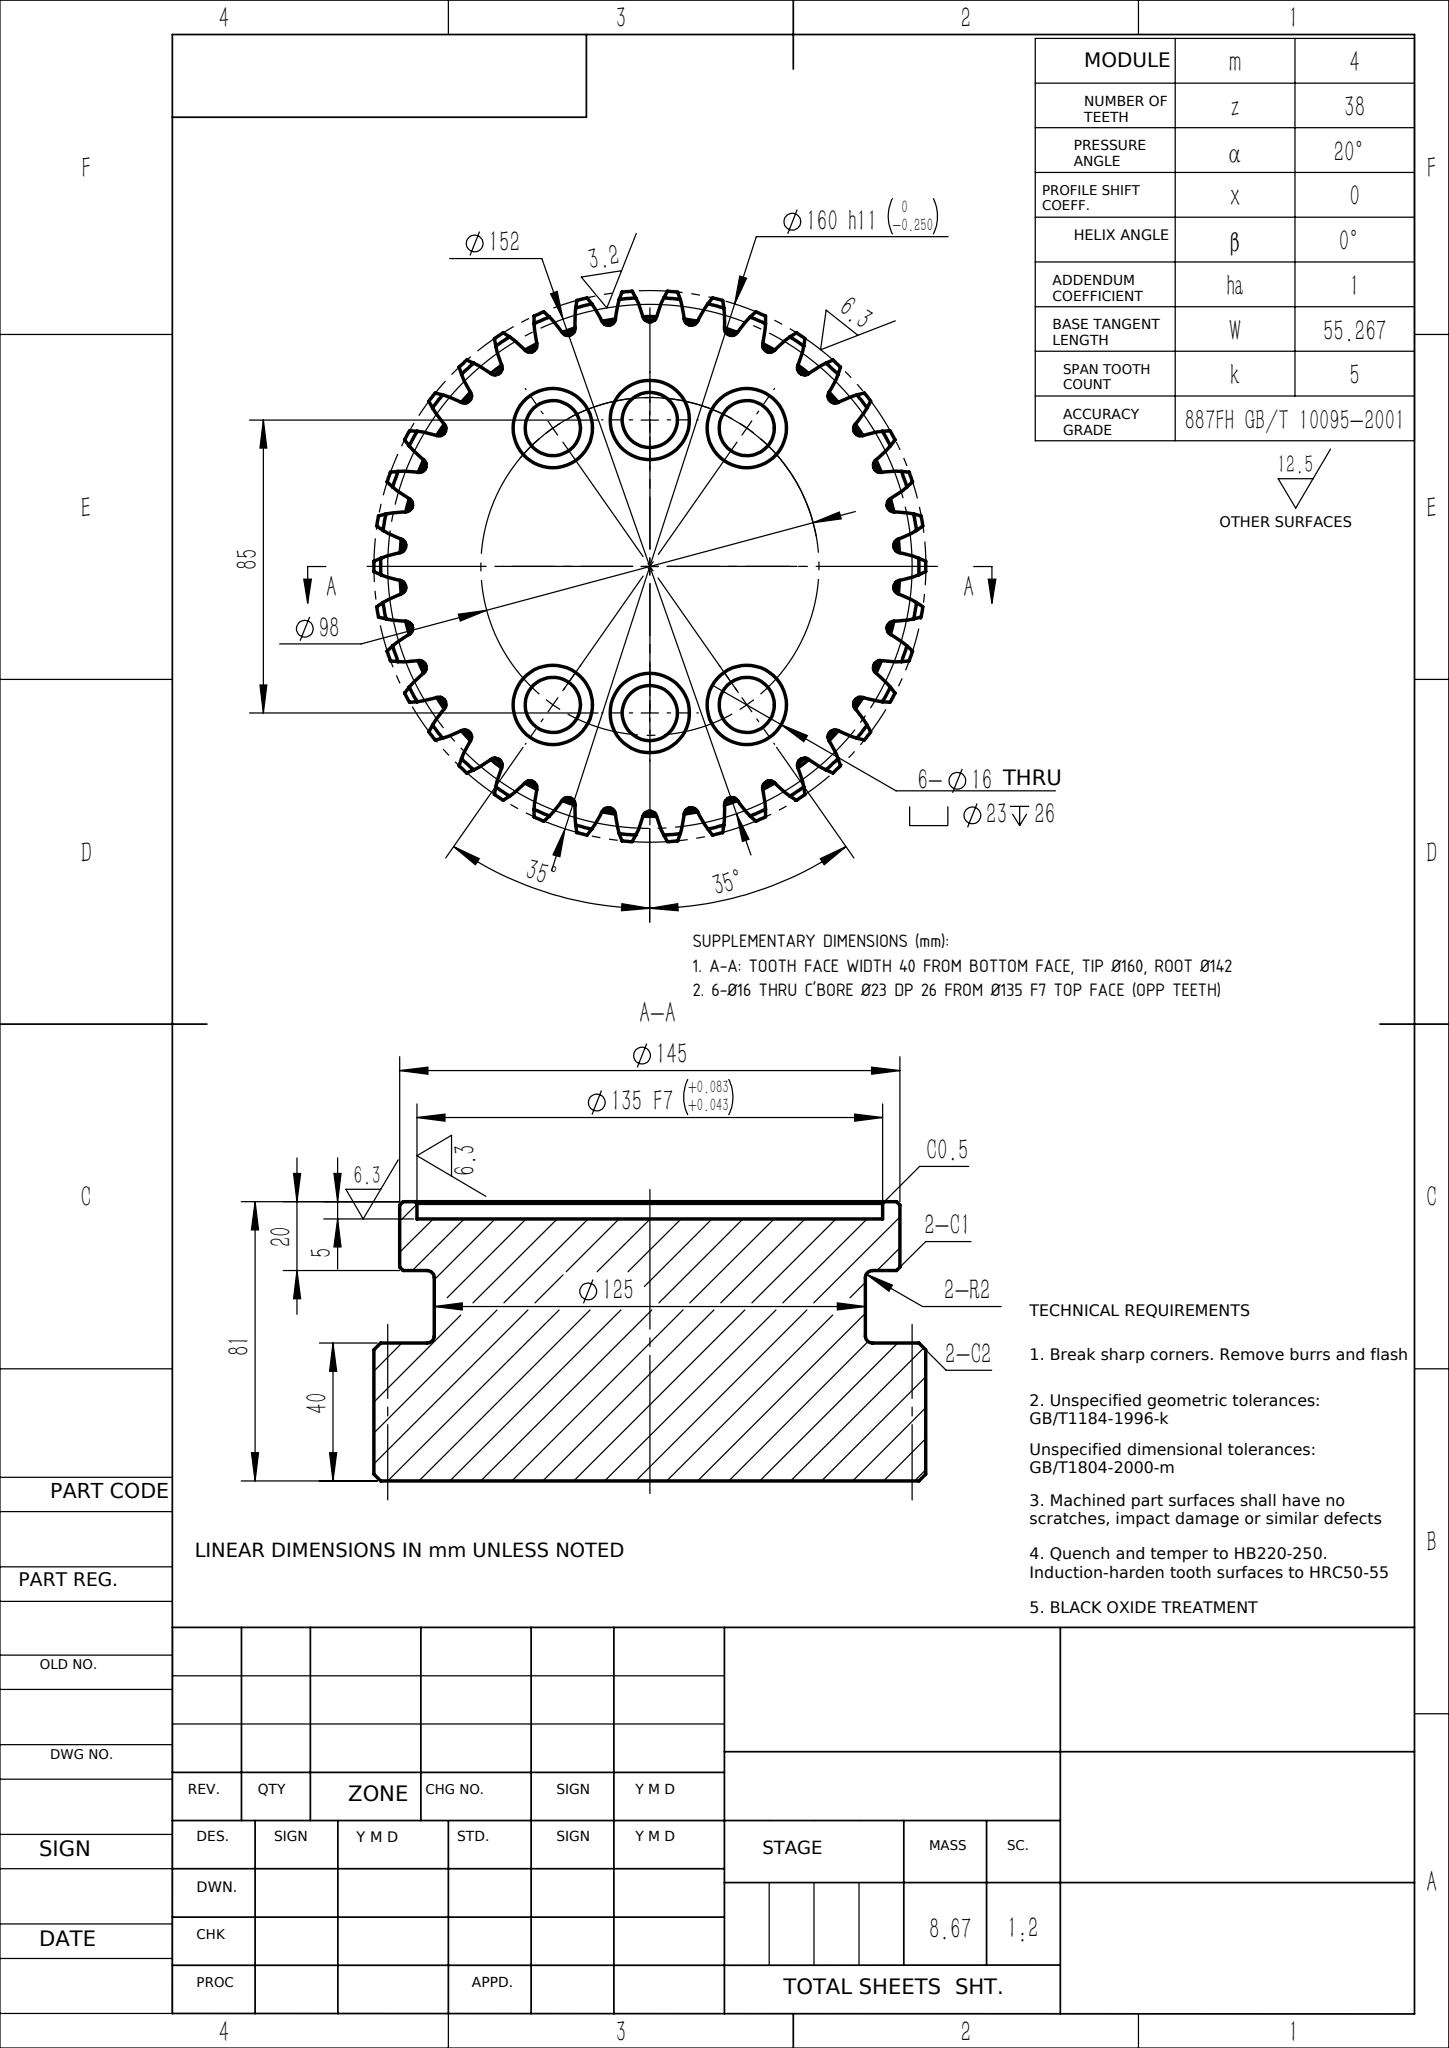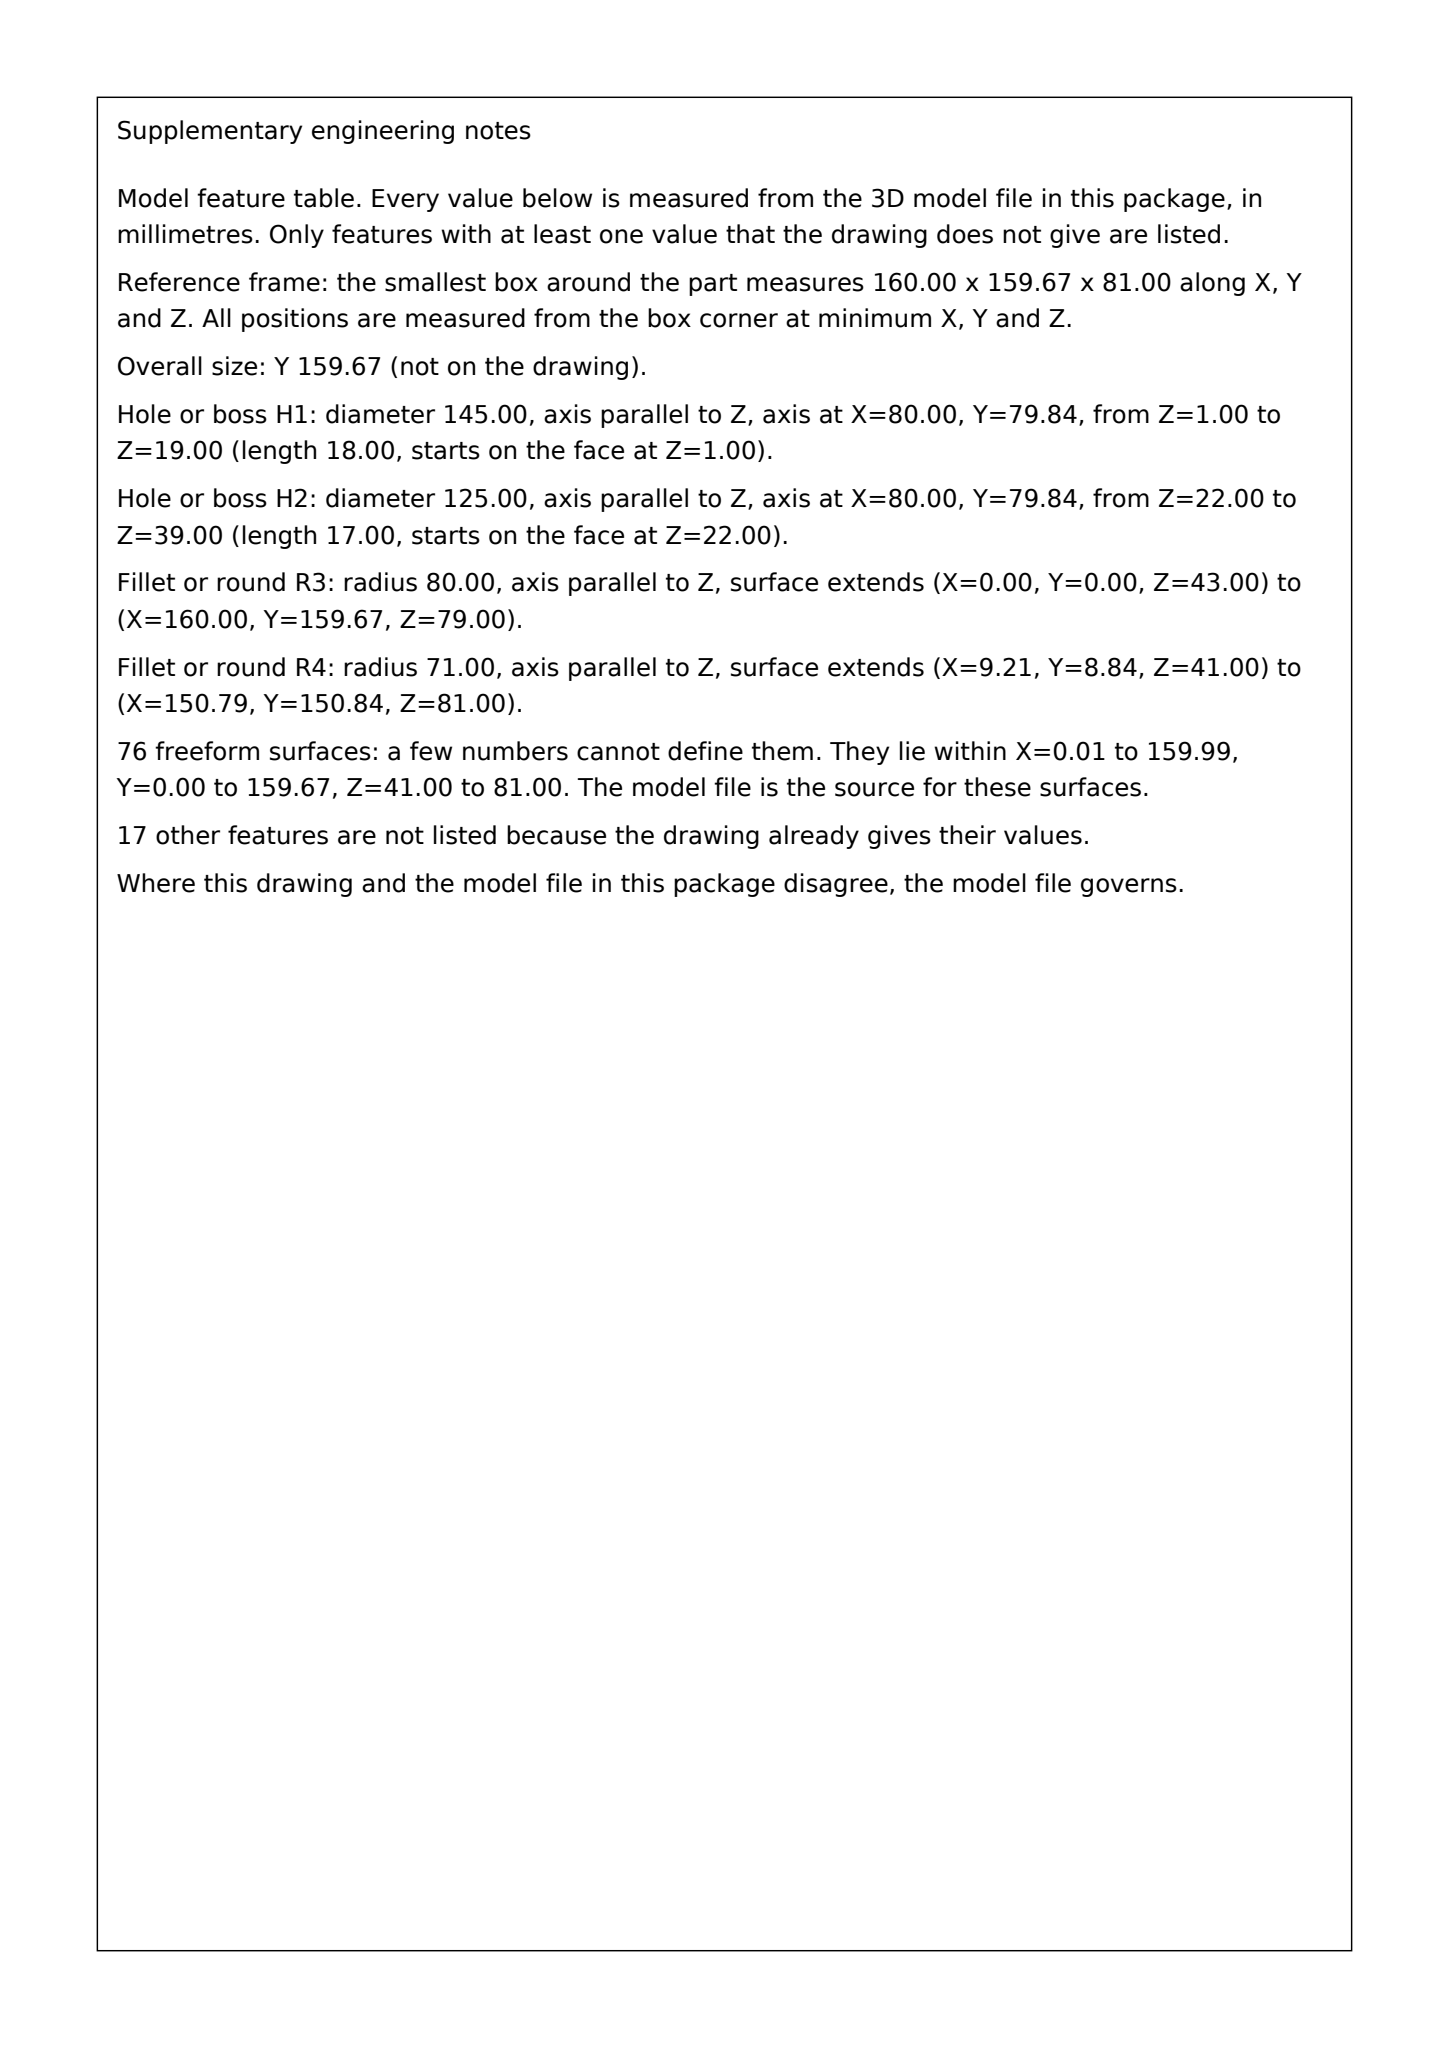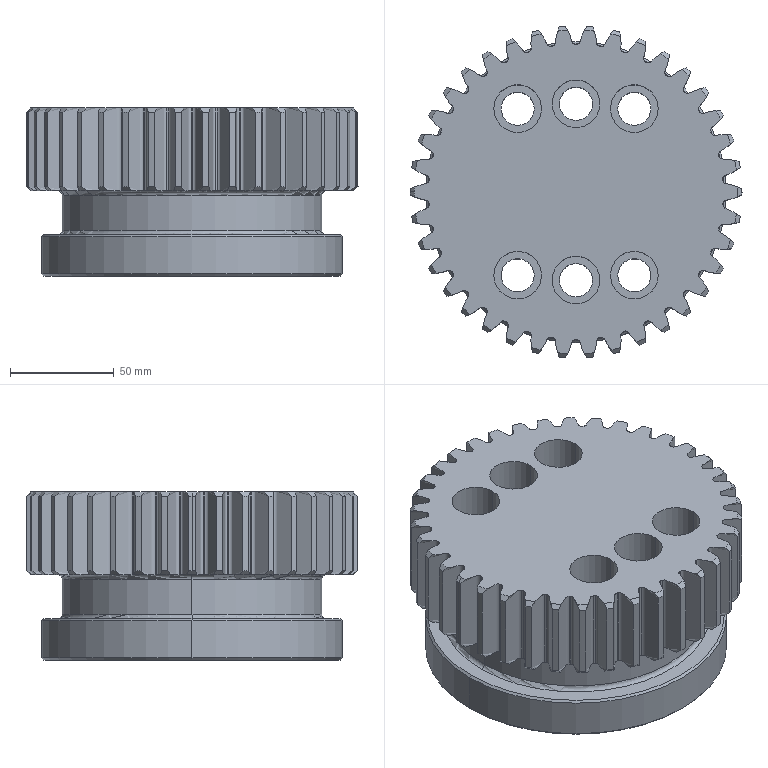Part | SolidWorks | mm | 1 solid | 282 faces | box 160 x 159.67 x 81 mm | volume 1111068 mm3 | cylinder 107 | cone 84 | spline 76 | plane 11 | torus 4 | commonest cylinder face diameters 160 x39 142 x38 23 x12 16 x12 135 x2 145 x2 125 x2